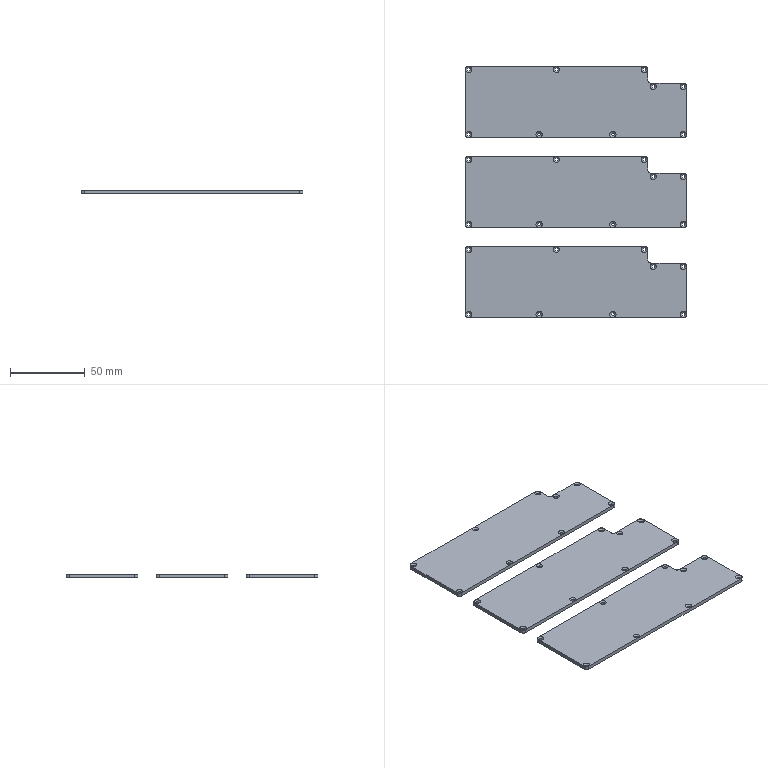CAM job | Mastercam | mm | 9 operations | part box 147.7 x 167.8 x 2.5
1. 2D High Speed (2D Area Mill) | 6 - 6 平铣刀
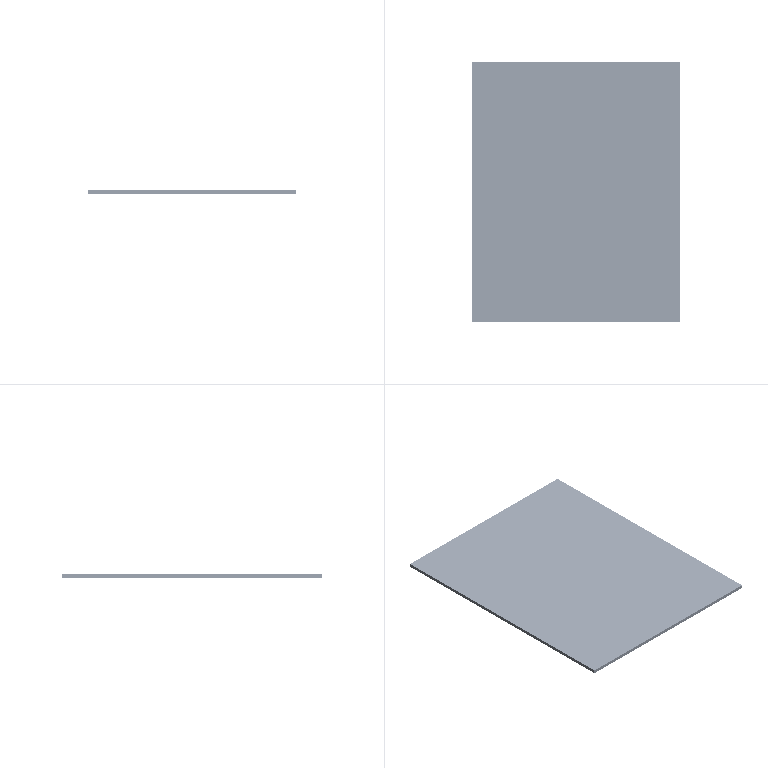2. Contour (Ramp) | 1 - 1 平铣刀
3. Contour (Remachining) | 3 - 3 平铣刀
4. 2D High Speed (2D Area Mill) | 3 - 3 平铣刀
5. Contour (2D) | 3 - 3 平铣刀
6. Contour (Ramp) | 3 - 3 平铣刀
7. Drill/Counterbore | 7 - 4 倒角刀
8. Contour (2D chamfer) | 7 - 4 倒角刀
9. Contour (2D) | 2 - 2 平铣刀